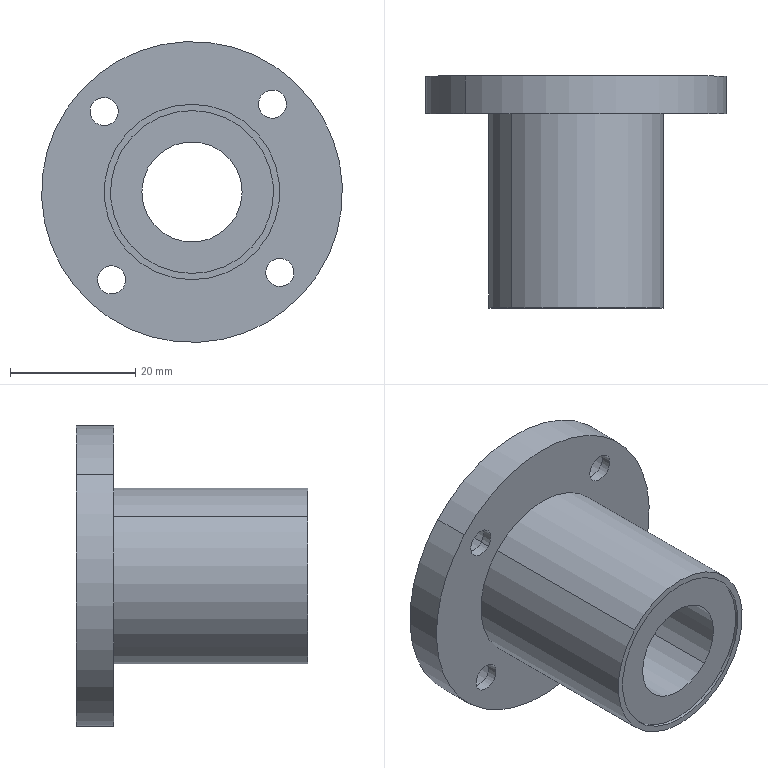Component | SolidWorks | LinearBearingSamickLMF16UU-5 | 1 solid | 38 faces | box 48 x 37 x 48 mm | volume 21132 mm3 | cylinder 28 | plane 10 | commonest cylinder face diameters 4.5 x8 8 x8 28 x4 26 x4 48 x2 16 x2
STEP:
#1=COLOUR_RGB('',0.7922,0.8196,0.9333);
#2=FILL_AREA_STYLE_COLOUR('',#1);
#3=FILL_AREA_STYLE('',(#2));
#4=SURFACE_STYLE_FILL_AREA(#3);
#5=SURFACE_SIDE_STYLE('',(#4));
#6=SURFACE_STYLE_USAGE(.BOTH.,#5);
#7=PRESENTATION_STYLE_ASSIGNMENT((#6));
#8=CARTESIAN_POINT('',(-6.706,-8.858,4.309));
#9=VERTEX_POINT('',#8);
#10=CARTESIAN_POINT('',(-5.893,-8.858,3.565));
#11=VERTEX_POINT('',#10);
#12=CARTESIAN_POINT('',(-6.299,-8.858,3.937));
#13=DIRECTION('',(0.,-1.,0.));
#14=DIRECTION('',(-0.7376,0.,0.6752));
#15=AXIS2_PLACEMENT_3D('',#12,#13,#14);
#16=CIRCLE('',#15,0.5512);
#17=EDGE_CURVE('',#9,#11,#16,.T.);
#18=ORIENTED_EDGE('',*,*,#17,.T.);
#19=CARTESIAN_POINT('',(-5.893,-10.079,3.565));
#20=VERTEX_POINT('',#19);
#21=CARTESIAN_POINT('',(-5.893,-8.622,3.565));
#22=DIRECTION('',(0.,-1.,0.));
#23=VECTOR('',#22,39.37);
#24=LINE('',#21,#23);
#25=EDGE_CURVE('',#11,#20,#24,.T.);
#26=ORIENTED_EDGE('',*,*,#25,.T.);
#27=CARTESIAN_POINT('',(-6.706,-10.079,4.309));
#28=VERTEX_POINT('',#27);
#29=CARTESIAN_POINT('',(-6.299,-10.079,3.937));
#30=DIRECTION('',(0.,1.,0.));
#31=DIRECTION('',(-0.7376,0.,0.6752));
#32=AXIS2_PLACEMENT_3D('',#29,#30,#31);
#33=CIRCLE('',#32,0.5512);
#34=EDGE_CURVE('',#20,#28,#33,.T.);
#35=ORIENTED_EDGE('',*,*,#34,.T.);
#36=CARTESIAN_POINT('',(-6.706,-8.622,4.309));
#37=DIRECTION('',(0.,-1.,0.));
#38=VECTOR('',#37,39.37);
#39=LINE('',#36,#38);
#40=EDGE_CURVE('',#9,#28,#39,.T.);
#41=ORIENTED_EDGE('',*,*,#40,.F.);
#42=EDGE_LOOP('',(#18,#26,#35,#41));
#43=FACE_OUTER_BOUND('',#42,.T.);
#44=CARTESIAN_POINT('',(-6.299,-8.622,3.937));
#45=DIRECTION('',(0.,-1.,0.));
#46=DIRECTION('',(-0.7376,0.,0.6752));
#47=AXIS2_PLACEMENT_3D('',#44,#45,#46);
#48=CYLINDRICAL_SURFACE('',#47,0.5512);
#49=ADVANCED_FACE('',(#43),#48,.T.);
#50=CARTESIAN_POINT('',(-5.922,-10.079,3.591));
#51=VERTEX_POINT('',#50);
#52=CARTESIAN_POINT('',(-6.677,-10.079,4.283));
#53=VERTEX_POINT('',#52);
#54=CARTESIAN_POINT('',(-6.299,-10.079,3.937));
#55=DIRECTION('',(0.,-1.,0.));
#56=DIRECTION('',(0.7376,0.,-0.6752));
#57=AXIS2_PLACEMENT_3D('',#54,#55,#56);
#58=CIRCLE('',#57,0.5118);
#59=EDGE_CURVE('',#51,#53,#58,.T.);
#60=ORIENTED_EDGE('',*,*,#59,.T.);
#61=CARTESIAN_POINT('',(-6.677,-10.059,4.283));
#62=VERTEX_POINT('',#61);
#63=CARTESIAN_POINT('',(-6.677,-10.079,4.283));
#64=DIRECTION('',(0.,1.,0.));
#65=VECTOR('',#64,39.37);
#66=LINE('',#63,#65);
#67=EDGE_CURVE('',#53,#62,#66,.T.);
#68=ORIENTED_EDGE('',*,*,#67,.T.);
#69=CARTESIAN_POINT('',(-5.922,-10.059,3.591));
#70=VERTEX_POINT('',#69);
#71=CARTESIAN_POINT('',(-6.299,-10.059,3.937));
#72=DIRECTION('',(0.,-1.,0.));
#73=DIRECTION('',(0.7376,0.,-0.6752));
#74=AXIS2_PLACEMENT_3D('',#71,#72,#73);
#75=CIRCLE('',#74,0.5118);
#76=EDGE_CURVE('',#70,#62,#75,.T.);
#77=ORIENTED_EDGE('',*,*,#76,.F.);
#78=CARTESIAN_POINT('',(-5.922,-10.079,3.591));
#79=DIRECTION('',(0.,1.,0.));
#80=VECTOR('',#79,39.37);
#81=LINE('',#78,#80);
#82=EDGE_CURVE('',#51,#70,#81,.T.);
#83=ORIENTED_EDGE('',*,*,#82,.F.);
#84=EDGE_LOOP('',(#60,#68,#77,#83));
#85=FACE_OUTER_BOUND('',#84,.T.);
#86=CARTESIAN_POINT('',(-6.299,-10.079,3.937));
#87=DIRECTION('',(0.,1.,0.));
#88=DIRECTION('',(0.7376,0.,-0.6752));
#89=AXIS2_PLACEMENT_3D('',#86,#87,#88);
#90=CYLINDRICAL_SURFACE('',#89,0.5118);
#91=ADVANCED_FACE('',(#85),#90,.F.);
#92=CARTESIAN_POINT('',(-6.864,-8.858,3.32));
#93=VERTEX_POINT('',#92);
#94=CARTESIAN_POINT('',(-6.744,-8.858,3.451));
#95=VERTEX_POINT('',#94);
#96=CARTESIAN_POINT('',(-6.804,-8.858,3.385));
#97=DIRECTION('',(0.,-1.,0.));
#98=DIRECTION('',(-0.6752,0.,-0.7376));
#99=AXIS2_PLACEMENT_3D('',#96,#97,#98);
#100=CIRCLE('',#99,0.08858);
#101=EDGE_CURVE('',#93,#95,#100,.T.);
#102=ORIENTED_EDGE('',*,*,#101,.T.);
#103=CARTESIAN_POINT('',(-6.744,-8.795,3.451));
#104=VERTEX_POINT('',#103);
#105=CARTESIAN_POINT('',(-6.744,-8.827,3.451));
#106=DIRECTION('',(-0.,1.,-0.));
#107=VECTOR('',#106,39.37);
#108=LINE('',#105,#107);
#109=EDGE_CURVE('',#95,#104,#108,.T.);
#110=ORIENTED_EDGE('',*,*,#109,.T.);
#111=CARTESIAN_POINT('',(-6.864,-8.795,3.32));
#112=VERTEX_POINT('',#111);
#113=CARTESIAN_POINT('',(-6.804,-8.795,3.385));
#114=DIRECTION('',(0.,-1.,0.));
#115=DIRECTION('',(-0.6752,0.,-0.7376));
#116=AXIS2_PLACEMENT_3D('',#113,#114,#115);
#117=CIRCLE('',#116,0.08858);
#118=EDGE_CURVE('',#112,#104,#117,.T.);
#119=ORIENTED_EDGE('',*,*,#118,.F.);
#120=CARTESIAN_POINT('',(-6.864,-8.827,3.32));
#121=DIRECTION('',(-0.,1.,-0.));
#122=VECTOR('',#121,39.37);
#123=LINE('',#120,#122);
#124=EDGE_CURVE('',#93,#112,#123,.T.);
#125=ORIENTED_EDGE('',*,*,#124,.F.);
#126=EDGE_LOOP('',(#102,#110,#119,#125));
#127=FACE_OUTER_BOUND('',#126,.T.);
#128=CARTESIAN_POINT('',(-6.804,-8.827,3.385));
#129=DIRECTION('',(-0.,1.,-0.));
#130=DIRECTION('',(-0.6752,0.,-0.7376));
#131=AXIS2_PLACEMENT_3D('',#128,#129,#130);
#132=CYLINDRICAL_SURFACE('',#131,0.08858);
#133=ADVANCED_FACE('',(#127),#132,.F.);
#134=CARTESIAN_POINT('',(-5.682,-8.858,3.372));
#135=VERTEX_POINT('',#134);
#136=CARTESIAN_POINT('',(-5.813,-8.858,3.492));
#137=VERTEX_POINT('',#136);
#138=CARTESIAN_POINT('',(-5.747,-8.858,3.432));
#139=DIRECTION('',(-0.,-1.,0.));
#140=DIRECTION('',(0.7376,0.,-0.6752));
#141=AXIS2_PLACEMENT_3D('',#138,#139,#140);
#142=CIRCLE('',#141,0.08858);
#143=EDGE_CURVE('',#135,#137,#142,.T.);
#144=ORIENTED_EDGE('',*,*,#143,.T.);
#145=CARTESIAN_POINT('',(-5.813,-8.795,3.492));
#146=VERTEX_POINT('',#145);
#147=CARTESIAN_POINT('',(-5.813,-8.827,3.492));
#148=DIRECTION('',(0.,1.,-0.));
#149=VECTOR('',#148,39.37);
#150=LINE('',#147,#149);
#151=EDGE_CURVE('',#137,#146,#150,.T.);
#152=ORIENTED_EDGE('',*,*,#151,.T.);
#153=CARTESIAN_POINT('',(-5.682,-8.795,3.372));
#154=VERTEX_POINT('',#153);
#155=CARTESIAN_POINT('',(-5.747,-8.795,3.432));
#156=DIRECTION('',(-0.,-1.,0.));
#157=DIRECTION('',(0.7376,0.,-0.6752));
#158=AXIS2_PLACEMENT_3D('',#155,#156,#157);
#159=CIRCLE('',#158,0.08858);
#160=EDGE_CURVE('',#154,#146,#159,.T.);
#161=ORIENTED_EDGE('',*,*,#160,.F.);
#162=CARTESIAN_POINT('',(-5.682,-8.827,3.372));
#163=DIRECTION('',(0.,1.,-0.));
#164=VECTOR('',#163,39.37);
#165=LINE('',#162,#164);
#166=EDGE_CURVE('',#135,#154,#165,.T.);
#167=ORIENTED_EDGE('',*,*,#166,.F.);
#168=EDGE_LOOP('',(#144,#152,#161,#167));
#169=FACE_OUTER_BOUND('',#168,.T.);
#170=CARTESIAN_POINT('',(-5.747,-8.827,3.432));
#171=DIRECTION('',(0.,1.,-0.));
#172=DIRECTION('',(0.7376,0.,-0.6752));
#173=AXIS2_PLACEMENT_3D('',#170,#171,#172);
#174=CYLINDRICAL_SURFACE('',#173,0.08858);
#175=ADVANCED_FACE('',(#169),#174,.F.);
#176=CARTESIAN_POINT('',(-5.854,-8.858,4.423));
#177=VERTEX_POINT('',#176);
#178=CARTESIAN_POINT('',(-5.734,-8.858,4.554));
#179=VERTEX_POINT('',#178);
#180=CARTESIAN_POINT('',(-5.794,-8.858,4.489));
#181=DIRECTION('',(-0.,-1.,-0.));
#182=DIRECTION('',(-0.6752,0.,-0.7376));
#183=AXIS2_PLACEMENT_3D('',#180,#181,#182);
#184=CIRCLE('',#183,0.08858);
#185=EDGE_CURVE('',#177,#179,#184,.T.);
#186=ORIENTED_EDGE('',*,*,#185,.T.);
#187=CARTESIAN_POINT('',(-5.734,-8.795,4.554));
#188=VERTEX_POINT('',#187);
#189=CARTESIAN_POINT('',(-5.734,-8.827,4.554));
#190=DIRECTION('',(0.,1.,0.));
#191=VECTOR('',#190,39.37);
#192=LINE('',#189,#191);
#193=EDGE_CURVE('',#179,#188,#192,.T.);
#194=ORIENTED_EDGE('',*,*,#193,.T.);
#195=CARTESIAN_POINT('',(-5.854,-8.795,4.423));
#196=VERTEX_POINT('',#195);
#197=CARTESIAN_POINT('',(-5.794,-8.795,4.489));
#198=DIRECTION('',(-0.,-1.,-0.));
#199=DIRECTION('',(-0.6752,0.,-0.7376));
#200=AXIS2_PLACEMENT_3D('',#197,#198,#199);
#201=CIRCLE('',#200,0.08858);
#202=EDGE_CURVE('',#196,#188,#201,.T.);
#203=ORIENTED_EDGE('',*,*,#202,.F.);
#204=CARTESIAN_POINT('',(-5.854,-8.827,4.423));
#205=DIRECTION('',(0.,1.,0.));
#206=VECTOR('',#205,39.37);
#207=LINE('',#204,#206);
#208=EDGE_CURVE('',#177,#196,#207,.T.);
#209=ORIENTED_EDGE('',*,*,#208,.F.);
#210=EDGE_LOOP('',(#186,#194,#203,#209));
#211=FACE_OUTER_BOUND('',#210,.T.);
#212=CARTESIAN_POINT('',(-5.794,-8.827,4.489));
#213=DIRECTION('',(0.,1.,0.));
#214=DIRECTION('',(-0.6752,0.,-0.7376));
#215=AXIS2_PLACEMENT_3D('',#212,#213,#214);
#216=CYLINDRICAL_SURFACE('',#215,0.08858);
#217=ADVANCED_FACE('',(#211),#216,.F.);
#218=CARTESIAN_POINT('',(-6.786,-8.858,4.382));
#219=VERTEX_POINT('',#218);
#220=CARTESIAN_POINT('',(-6.916,-8.858,4.502));
#221=VERTEX_POINT('',#220);
#222=CARTESIAN_POINT('',(-6.851,-8.858,4.442));
#223=DIRECTION('',(0.,-1.,-0.));
#224=DIRECTION('',(0.7376,0.,-0.6752));
#225=AXIS2_PLACEMENT_3D('',#222,#223,#224);
#226=CIRCLE('',#225,0.08858);
#227=EDGE_CURVE('',#219,#221,#226,.T.);
#228=ORIENTED_EDGE('',*,*,#227,.T.);
#229=CARTESIAN_POINT('',(-6.916,-8.795,4.502));
#230=VERTEX_POINT('',#229);
#231=CARTESIAN_POINT('',(-6.916,-8.827,4.502));
#232=DIRECTION('',(-0.,1.,0.));
#233=VECTOR('',#232,39.37);
#234=LINE('',#231,#233);
#235=EDGE_CURVE('',#221,#230,#234,.T.);
#236=ORIENTED_EDGE('',*,*,#235,.T.);
#237=CARTESIAN_POINT('',(-6.786,-8.795,4.382));
#238=VERTEX_POINT('',#237);
#239=CARTESIAN_POINT('',(-6.851,-8.795,4.442));
#240=DIRECTION('',(0.,-1.,-0.));
#241=DIRECTION('',(0.7376,0.,-0.6752));
#242=AXIS2_PLACEMENT_3D('',#239,#240,#241);
#243=CIRCLE('',#242,0.08858);
#244=EDGE_CURVE('',#238,#230,#243,.T.);
#245=ORIENTED_EDGE('',*,*,#244,.F.);
#246=CARTESIAN_POINT('',(-6.786,-8.827,4.382));
#247=DIRECTION('',(-0.,1.,0.));
#248=VECTOR('',#247,39.37);
#249=LINE('',#246,#248);
#250=EDGE_CURVE('',#219,#238,#249,.T.);
#251=ORIENTED_EDGE('',*,*,#250,.F.);
#252=EDGE_LOOP('',(#228,#236,#245,#251));
#253=FACE_OUTER_BOUND('',#252,.T.);
#254=CARTESIAN_POINT('',(-6.851,-8.827,4.442));
#255=DIRECTION('',(-0.,1.,0.));
#256=DIRECTION('',(0.7376,0.,-0.6752));
#257=AXIS2_PLACEMENT_3D('',#254,#255,#256);
#258=CYLINDRICAL_SURFACE('',#257,0.08858);
#259=ADVANCED_FACE('',(#253),#258,.F.);
#260=CARTESIAN_POINT('',(-6.996,-8.622,4.575));
#261=VERTEX_POINT('',#260);
#262=CARTESIAN_POINT('',(-5.602,-8.622,3.299));
#263=VERTEX_POINT('',#262);
#264=CARTESIAN_POINT('',(-6.299,-8.622,3.937));
#265=DIRECTION('',(0.,-1.,0.));
#266=DIRECTION('',(-0.7376,0.,0.6752));
#267=AXIS2_PLACEMENT_3D('',#264,#265,#266);
#268=CIRCLE('',#267,0.9449);
#269=EDGE_CURVE('',#261,#263,#268,.T.);
#270=ORIENTED_EDGE('',*,*,#269,.T.);
#271=CARTESIAN_POINT('',(-5.602,-8.858,3.299));
#272=VERTEX_POINT('',#271);
#273=CARTESIAN_POINT('',(-5.602,-8.622,3.299));
#274=DIRECTION('',(0.,-1.,0.));
#275=VECTOR('',#274,39.37);
#276=LINE('',#273,#275);
#277=EDGE_CURVE('',#263,#272,#276,.T.);
#278=ORIENTED_EDGE('',*,*,#277,.T.);
#279=CARTESIAN_POINT('',(-6.996,-8.858,4.575));
#280=VERTEX_POINT('',#279);
#281=CARTESIAN_POINT('',(-6.299,-8.858,3.937));
#282=DIRECTION('',(0.,1.,0.));
#283=DIRECTION('',(-0.7376,0.,0.6752));
#284=AXIS2_PLACEMENT_3D('',#281,#282,#283);
#285=CIRCLE('',#284,0.9449);
#286=EDGE_CURVE('',#272,#280,#285,.T.);
#287=ORIENTED_EDGE('',*,*,#286,.T.);
#288=CARTESIAN_POINT('',(-6.996,-8.622,4.575));
#289=DIRECTION('',(0.,-1.,0.));
#290=VECTOR('',#289,39.37);
#291=LINE('',#288,#290);
#292=EDGE_CURVE('',#261,#280,#291,.T.);
#293=ORIENTED_EDGE('',*,*,#292,.F.);
#294=EDGE_LOOP('',(#270,#278,#287,#293));
#295=FACE_OUTER_BOUND('',#294,.T.);
#296=CARTESIAN_POINT('',(-6.299,-8.622,3.937));
#297=DIRECTION('',(0.,-1.,0.));
#298=DIRECTION('',(-0.7376,0.,0.6752));
#299=AXIS2_PLACEMENT_3D('',#296,#297,#298);
#300=CYLINDRICAL_SURFACE('',#299,0.9449);
#301=ADVANCED_FACE('',(#295),#300,.T.);
#302=CARTESIAN_POINT('',(-6.067,-8.646,3.724));
#303=VERTEX_POINT('',#302);
#304=CARTESIAN_POINT('',(-6.532,-8.646,4.15));
#305=VERTEX_POINT('',#304);
#306=CARTESIAN_POINT('',(-6.299,-8.646,3.937));
#307=DIRECTION('',(0.,-1.,0.));
#308=DIRECTION('',(-0.7376,0.,0.6752));
#309=AXIS2_PLACEMENT_3D('',#306,#307,#308);
#310=CIRCLE('',#309,0.315);
#311=EDGE_CURVE('',#303,#305,#310,.T.);
#312=ORIENTED_EDGE('',*,*,#311,.F.);
#313=CARTESIAN_POINT('',(-6.067,-10.059,3.724));
#314=VERTEX_POINT('',#313);
#315=CARTESIAN_POINT('',(-6.067,-8.622,3.724));
#316=DIRECTION('',(0.,-1.,0.));
#317=VECTOR('',#316,39.37);
#318=LINE('',#315,#317);
#319=EDGE_CURVE('',#303,#314,#318,.T.);
#320=ORIENTED_EDGE('',*,*,#319,.T.);
#321=CARTESIAN_POINT('',(-6.532,-10.059,4.15));
#322=VERTEX_POINT('',#321);
#323=CARTESIAN_POINT('',(-6.299,-10.059,3.937));
#324=DIRECTION('',(0.,-1.,0.));
#325=DIRECTION('',(-0.7376,0.,0.6752));
#326=AXIS2_PLACEMENT_3D('',#323,#324,#325);
#327=CIRCLE('',#326,0.315);
#328=EDGE_CURVE('',#314,#322,#327,.T.);
#329=ORIENTED_EDGE('',*,*,#328,.T.);
#330=CARTESIAN_POINT('',(-6.532,-8.622,4.15));
#331=DIRECTION('',(0.,-1.,0.));
#332=VECTOR('',#331,39.37);
#333=LINE('',#330,#332);
#334=EDGE_CURVE('',#305,#322,#333,.T.);
#335=ORIENTED_EDGE('',*,*,#334,.F.);
#336=EDGE_LOOP('',(#312,#320,#329,#335));
#337=FACE_OUTER_BOUND('',#336,.T.);
#338=CARTESIAN_POINT('',(-6.299,-8.622,3.937));
#339=DIRECTION('',(0.,-1.,0.));
#340=DIRECTION('',(-0.7376,0.,0.6752));
#341=AXIS2_PLACEMENT_3D('',#338,#339,#340);
#342=CYLINDRICAL_SURFACE('',#341,0.315);
#343=ADVANCED_FACE('',(#337),#342,.F.);
#344=CARTESIAN_POINT('',(-6.911,-8.795,3.269));
#345=VERTEX_POINT('',#344);
#346=CARTESIAN_POINT('',(-6.698,-8.795,3.501));
#347=VERTEX_POINT('',#346);
#348=CARTESIAN_POINT('',(-6.804,-8.795,3.385));
#349=DIRECTION('',(0.,-1.,0.));
#350=DIRECTION('',(-0.6752,0.,-0.7376));
#351=AXIS2_PLACEMENT_3D('',#348,#349,#350);
#352=CIRCLE('',#351,0.1575);
#353=EDGE_CURVE('',#345,#347,#352,.T.);
#354=ORIENTED_EDGE('',*,*,#353,.T.);
#355=CARTESIAN_POINT('',(-6.698,-8.622,3.501));
#356=VERTEX_POINT('',#355);
#357=CARTESIAN_POINT('',(-6.698,-8.709,3.501));
#358=DIRECTION('',(-0.,1.,-0.));
#359=VECTOR('',#358,39.37);
#360=LINE('',#357,#359);
#361=EDGE_CURVE('',#347,#356,#360,.T.);
#362=ORIENTED_EDGE('',*,*,#361,.T.);
#363=CARTESIAN_POINT('',(-6.911,-8.622,3.269));
#364=VERTEX_POINT('',#363);
#365=CARTESIAN_POINT('',(-6.804,-8.622,3.385));
#366=DIRECTION('',(0.,-1.,0.));
#367=DIRECTION('',(-0.6752,0.,-0.7376));
#368=AXIS2_PLACEMENT_3D('',#365,#366,#367);
#369=CIRCLE('',#368,0.1575);
#370=EDGE_CURVE('',#364,#356,#369,.T.);
#371=ORIENTED_EDGE('',*,*,#370,.F.);
#372=CARTESIAN_POINT('',(-6.911,-8.709,3.269));
#373=DIRECTION('',(-0.,1.,-0.));
#374=VECTOR('',#373,39.37);
#375=LINE('',#372,#374);
#376=EDGE_CURVE('',#345,#364,#375,.T.);
#377=ORIENTED_EDGE('',*,*,#376,.F.);
#378=EDGE_LOOP('',(#354,#362,#371,#377));
#379=FACE_OUTER_BOUND('',#378,.T.);
#380=CARTESIAN_POINT('',(-6.804,-8.709,3.385));
#381=DIRECTION('',(-0.,1.,-0.));
#382=DIRECTION('',(-0.6752,0.,-0.7376));
#383=AXIS2_PLACEMENT_3D('',#380,#381,#382);
#384=CYLINDRICAL_SURFACE('',#383,0.1575);
#385=ADVANCED_FACE('',(#379),#384,.F.);
#386=CARTESIAN_POINT('',(-5.631,-8.795,3.326));
#387=VERTEX_POINT('',#386);
#388=CARTESIAN_POINT('',(-5.864,-8.795,3.538));
#389=VERTEX_POINT('',#388);
#390=CARTESIAN_POINT('',(-5.747,-8.795,3.432));
#391=DIRECTION('',(-0.,-1.,0.));
#392=DIRECTION('',(0.7376,0.,-0.6752));
#393=AXIS2_PLACEMENT_3D('',#390,#391,#392);
#394=CIRCLE('',#393,0.1575);
#395=EDGE_CURVE('',#387,#389,#394,.T.);
#396=ORIENTED_EDGE('',*,*,#395,.T.);
#397=CARTESIAN_POINT('',(-5.864,-8.622,3.538));
#398=VERTEX_POINT('',#397);
#399=CARTESIAN_POINT('',(-5.864,-8.709,3.538));
#400=DIRECTION('',(0.,1.,-0.));
#401=VECTOR('',#400,39.37);
#402=LINE('',#399,#401);
#403=EDGE_CURVE('',#389,#398,#402,.T.);
#404=ORIENTED_EDGE('',*,*,#403,.T.);
#405=CARTESIAN_POINT('',(-5.631,-8.622,3.326));
#406=VERTEX_POINT('',#405);
#407=CARTESIAN_POINT('',(-5.747,-8.622,3.432));
#408=DIRECTION('',(-0.,-1.,0.));
#409=DIRECTION('',(0.7376,0.,-0.6752));
#410=AXIS2_PLACEMENT_3D('',#407,#408,#409);
#411=CIRCLE('',#410,0.1575);
#412=EDGE_CURVE('',#406,#398,#411,.T.);
#413=ORIENTED_EDGE('',*,*,#412,.F.);
#414=CARTESIAN_POINT('',(-5.631,-8.709,3.326));
#415=DIRECTION('',(0.,1.,-0.));
#416=VECTOR('',#415,39.37);
#417=LINE('',#414,#416);
#418=EDGE_CURVE('',#387,#406,#417,.T.);
#419=ORIENTED_EDGE('',*,*,#418,.F.);
#420=EDGE_LOOP('',(#396,#404,#413,#419));
#421=FACE_OUTER_BOUND('',#420,.T.);
#422=CARTESIAN_POINT('',(-5.747,-8.709,3.432));
#423=DIRECTION('',(0.,1.,-0.));
#424=DIRECTION('',(0.7376,0.,-0.6752));
#425=AXIS2_PLACEMENT_3D('',#422,#423,#424);
#426=CYLINDRICAL_SURFACE('',#425,0.1575);
#427=ADVANCED_FACE('',(#421),#426,.F.);
#428=CARTESIAN_POINT('',(-5.9,-8.795,4.373));
#429=VERTEX_POINT('',#428);
#430=CARTESIAN_POINT('',(-5.688,-8.795,4.605));
#431=VERTEX_POINT('',#430);
#432=CARTESIAN_POINT('',(-5.794,-8.795,4.489));
#433=DIRECTION('',(-0.,-1.,-0.));
#434=DIRECTION('',(-0.6752,0.,-0.7376));
#435=AXIS2_PLACEMENT_3D('',#432,#433,#434);
#436=CIRCLE('',#435,0.1575);
#437=EDGE_CURVE('',#429,#431,#436,.T.);
#438=ORIENTED_EDGE('',*,*,#437,.T.);
#439=CARTESIAN_POINT('',(-5.688,-8.622,4.605));
#440=VERTEX_POINT('',#439);
#441=CARTESIAN_POINT('',(-5.688,-8.709,4.605));
#442=DIRECTION('',(0.,1.,0.));
#443=VECTOR('',#442,39.37);
#444=LINE('',#441,#443);
#445=EDGE_CURVE('',#431,#440,#444,.T.);
#446=ORIENTED_EDGE('',*,*,#445,.T.);
#447=CARTESIAN_POINT('',(-5.9,-8.622,4.373));
#448=VERTEX_POINT('',#447);
#449=CARTESIAN_POINT('',(-5.794,-8.622,4.489));
#450=DIRECTION('',(-0.,-1.,-0.));
#451=DIRECTION('',(-0.6752,0.,-0.7376));
#452=AXIS2_PLACEMENT_3D('',#449,#450,#451);
#453=CIRCLE('',#452,0.1575);
#454=EDGE_CURVE('',#448,#440,#453,.T.);
#455=ORIENTED_EDGE('',*,*,#454,.F.);
#456=CARTESIAN_POINT('',(-5.9,-8.709,4.373));
#457=DIRECTION('',(0.,1.,0.));
#458=VECTOR('',#457,39.37);
#459=LINE('',#456,#458);
#460=EDGE_CURVE('',#429,#448,#459,.T.);
#461=ORIENTED_EDGE('',*,*,#460,.F.);
#462=EDGE_LOOP('',(#438,#446,#455,#461));
#463=FACE_OUTER_BOUND('',#462,.T.);
#464=CARTESIAN_POINT('',(-5.794,-8.709,4.489));
#465=DIRECTION('',(0.,1.,0.));
#466=DIRECTION('',(-0.6752,0.,-0.7376));
#467=AXIS2_PLACEMENT_3D('',#464,#465,#466);
#468=CYLINDRICAL_SURFACE('',#467,0.1575);
#469=ADVANCED_FACE('',(#463),#468,.F.);
#470=CARTESIAN_POINT('',(-6.735,-8.795,4.336));
#471=VERTEX_POINT('',#470);
#472=CARTESIAN_POINT('',(-6.967,-8.795,4.548));
#473=VERTEX_POINT('',#472);
#474=CARTESIAN_POINT('',(-6.851,-8.795,4.442));
#475=DIRECTION('',(0.,-1.,-0.));
#476=DIRECTION('',(0.7376,0.,-0.6752));
#477=AXIS2_PLACEMENT_3D('',#474,#475,#476);
#478=CIRCLE('',#477,0.1575);
#479=EDGE_CURVE('',#471,#473,#478,.T.);
#480=ORIENTED_EDGE('',*,*,#479,.T.);
#481=CARTESIAN_POINT('',(-6.967,-8.622,4.548));
#482=VERTEX_POINT('',#481);
#483=CARTESIAN_POINT('',(-6.967,-8.709,4.548));
#484=DIRECTION('',(-0.,1.,0.));
#485=VECTOR('',#484,39.37);
#486=LINE('',#483,#485);
#487=EDGE_CURVE('',#473,#482,#486,.T.);
#488=ORIENTED_EDGE('',*,*,#487,.T.);
#489=CARTESIAN_POINT('',(-6.735,-8.622,4.336));
#490=VERTEX_POINT('',#489);
#491=CARTESIAN_POINT('',(-6.851,-8.622,4.442));
#492=DIRECTION('',(0.,-1.,-0.));
#493=DIRECTION('',(0.7376,0.,-0.6752));
#494=AXIS2_PLACEMENT_3D('',#491,#492,#493);
#495=CIRCLE('',#494,0.1575);
#496=EDGE_CURVE('',#490,#482,#495,.T.);
#497=ORIENTED_EDGE('',*,*,#496,.F.);
#498=CARTESIAN_POINT('',(-6.735,-8.709,4.336));
#499=DIRECTION('',(-0.,1.,0.));
#500=VECTOR('',#499,39.37);
#501=LINE('',#498,#500);
#502=EDGE_CURVE('',#471,#490,#501,.T.);
#503=ORIENTED_EDGE('',*,*,#502,.F.);
#504=EDGE_LOOP('',(#480,#488,#497,#503));
#505=FACE_OUTER_BOUND('',#504,.T.);
#506=CARTESIAN_POINT('',(-6.851,-8.709,4.442));
#507=DIRECTION('',(-0.,1.,0.));
#508=DIRECTION('',(0.7376,0.,-0.6752));
#509=AXIS2_PLACEMENT_3D('',#506,#507,#508);
#510=CYLINDRICAL_SURFACE('',#509,0.1575);
#511=ADVANCED_FACE('',(#505),#510,.F.);
#512=CARTESIAN_POINT('',(-5.893,-8.622,3.565));
#513=VERTEX_POINT('',#512);
#514=CARTESIAN_POINT('',(-6.706,-8.622,4.309));
#515=VERTEX_POINT('',#514);
#516=CARTESIAN_POINT('',(-6.299,-8.622,3.937));
#517=DIRECTION('',(0.,-1.,0.));
#518=DIRECTION('',(-0.7376,0.,0.6752));
#519=AXIS2_PLACEMENT_3D('',#516,#517,#518);
#520=CIRCLE('',#519,0.5512);
#521=EDGE_CURVE('',#513,#515,#520,.T.);
#522=ORIENTED_EDGE('',*,*,#521,.F.);
#523=CARTESIAN_POINT('',(-5.893,-8.634,3.565));
#524=VERTEX_POINT('',#523);
#525=CARTESIAN_POINT('',(-5.893,-8.622,3.565));
#526=DIRECTION('',(0.,-1.,0.));
#527=VECTOR('',#526,39.37);
#528=LINE('',#525,#527);
#529=EDGE_CURVE('',#513,#524,#528,.T.);
#530=ORIENTED_EDGE('',*,*,#529,.T.);
#531=CARTESIAN_POINT('',(-6.706,-8.634,4.309));
#532=VERTEX_POINT('',#531);
#533=CARTESIAN_POINT('',(-6.299,-8.634,3.937));
#534=DIRECTION('',(0.,1.,0.));
#535=DIRECTION('',(-0.7376,0.,0.6752));
#536=AXIS2_PLACEMENT_3D('',#533,#534,#535);
#537=CIRCLE('',#536,0.5512);
#538=EDGE_CURVE('',#532,#524,#537,.T.);
#539=ORIENTED_EDGE('',*,*,#538,.F.);
#540=CARTESIAN_POINT('',(-6.706,-8.622,4.309));
#541=DIRECTION('',(0.,-1.,0.));
#542=VECTOR('',#541,39.37);
#543=LINE('',#540,#542);
#544=EDGE_CURVE('',#515,#532,#543,.T.);
#545=ORIENTED_EDGE('',*,*,#544,.F.);
#546=EDGE_LOOP('',(#522,#530,#539,#545));
#547=FACE_OUTER_BOUND('',#546,.T.);
#548=CARTESIAN_POINT('',(-6.299,-8.622,3.937));
#549=DIRECTION('',(0.,-1.,0.));
#550=DIRECTION('',(-0.7376,0.,0.6752));
#551=AXIS2_PLACEMENT_3D('',#548,#549,#550);
#552=CYLINDRICAL_SURFACE('',#551,0.5512);
#553=ADVANCED_FACE('',(#547),#552,.F.);
#554=CARTESIAN_POINT('',(-5.922,-8.634,3.591));
#555=VERTEX_POINT('',#554);
#556=CARTESIAN_POINT('',(-6.677,-8.634,4.283));
#557=VERTEX_POINT('',#556);
#558=CARTESIAN_POINT('',(-6.299,-8.634,3.937));
#559=DIRECTION('',(0.,-1.,0.));
#560=DIRECTION('',(-0.7376,0.,0.6752));
#561=AXIS2_PLACEMENT_3D('',#558,#559,#560);
#562=CIRCLE('',#561,0.5118);
#563=EDGE_CURVE('',#555,#557,#562,.T.);
#564=ORIENTED_EDGE('',*,*,#563,.F.);
#565=CARTESIAN_POINT('',(-5.922,-8.646,3.591));
#566=VERTEX_POINT('',#565);
#567=CARTESIAN_POINT('',(-5.922,-8.622,3.591));
#568=DIRECTION('',(0.,-1.,0.));
#569=VECTOR('',#568,39.37);
#570=LINE('',#567,#569);
#571=EDGE_CURVE('',#555,#566,#570,.T.);
#572=ORIENTED_EDGE('',*,*,#571,.T.);
#573=CARTESIAN_POINT('',(-6.677,-8.646,4.283));
#574=VERTEX_POINT('',#573);
#575=CARTESIAN_POINT('',(-6.299,-8.646,3.937));
#576=DIRECTION('',(0.,1.,0.));
#577=DIRECTION('',(-0.7376,0.,0.6752));
#578=AXIS2_PLACEMENT_3D('',#575,#576,#577);
#579=CIRCLE('',#578,0.5118);
#580=EDGE_CURVE('',#574,#566,#579,.T.);
#581=ORIENTED_EDGE('',*,*,#580,.F.);
#582=CARTESIAN_POINT('',(-6.677,-8.622,4.283));
#583=DIRECTION('',(0.,-1.,0.));
#584=VECTOR('',#583,39.37);
#585=LINE('',#582,#584);
#586=EDGE_CURVE('',#557,#574,#585,.T.);
#587=ORIENTED_EDGE('',*,*,#586,.F.);
#588=EDGE_LOOP('',(#564,#572,#581,#587));
#589=FACE_OUTER_BOUND('',#588,.T.);
#590=CARTESIAN_POINT('',(-6.299,-8.622,3.937));
#591=DIRECTION('',(0.,-1.,0.));
#592=DIRECTION('',(-0.7376,0.,0.6752));
#593=AXIS2_PLACEMENT_3D('',#590,#591,#592);
#594=CYLINDRICAL_SURFACE('',#593,0.5118);
#595=ADVANCED_FACE('',(#589),#594,.F.);
#596=ORIENTED_EDGE('',*,*,#25,.F.);
#597=CARTESIAN_POINT('',(-6.299,-8.858,3.937));
#598=DIRECTION('',(0.,-1.,0.));
#599=DIRECTION('',(-0.7376,0.,0.6752));
#600=AXIS2_PLACEMENT_3D('',#597,#598,#599);
#601=CIRCLE('',#600,0.5512);
#602=EDGE_CURVE('',#11,#9,#601,.T.);
#603=ORIENTED_EDGE('',*,*,#602,.T.);
#604=ORIENTED_EDGE('',*,*,#40,.T.);
#605=CARTESIAN_POINT('',(-6.299,-10.079,3.937));
#606=DIRECTION('',(0.,1.,0.));
#607=DIRECTION('',(-0.7376,0.,0.6752));
#608=AXIS2_PLACEMENT_3D('',#605,#606,#607);
#609=CIRCLE('',#608,0.5512);
#610=EDGE_CURVE('',#28,#20,#609,.T.);
#611=ORIENTED_EDGE('',*,*,#610,.T.);
#612=EDGE_LOOP('',(#596,#603,#604,#611));
#613=FACE_OUTER_BOUND('',#612,.T.);
#614=CARTESIAN_POINT('',(-6.299,-8.622,3.937));
#615=DIRECTION('',(0.,-1.,0.));
#616=DIRECTION('',(-0.7376,0.,0.6752));
#617=AXIS2_PLACEMENT_3D('',#614,#615,#616);
#618=CYLINDRICAL_SURFACE('',#617,0.5512);
#619=ADVANCED_FACE('',(#613),#618,.T.);
#620=ORIENTED_EDGE('',*,*,#59,.F.);
#621=CARTESIAN_POINT('',(-6.299,-10.079,3.937));
#622=DIRECTION('',(0.,-1.,0.));
#623=DIRECTION('',(0.7376,0.,-0.6752));
#624=AXIS2_PLACEMENT_3D('',#621,#622,#623);
#625=CIRCLE('',#624,0.5118);
#626=EDGE_CURVE('',#53,#51,#625,.T.);
#627=ORIENTED_EDGE('',*,*,#626,.F.);
#628=EDGE_LOOP('',(#620,#627));
#629=FACE_BOUND('',#628,.T.);
#630=ORIENTED_EDGE('',*,*,#610,.F.);
#631=ORIENTED_EDGE('',*,*,#34,.F.);
#632=EDGE_LOOP('',(#630,#631));
#633=FACE_OUTER_BOUND('',#632,.T.);
#634=CARTESIAN_POINT('',(-6.299,-10.079,3.937));
#635=DIRECTION('',(0.,1.,0.));
#636=DIRECTION('',(0.7376,0.,-0.6752));
#637=AXIS2_PLACEMENT_3D('',#634,#635,#636);
#638=PLANE('',#637);
#639=ADVANCED_FACE('',(#629,#633),#638,.F.);
#640=ORIENTED_EDGE('',*,*,#17,.F.);
#641=ORIENTED_EDGE('',*,*,#602,.F.);
#642=EDGE_LOOP('',(#640,#641));
#643=FACE_BOUND('',#642,.T.);
#644=ORIENTED_EDGE('',*,*,#101,.F.);
#645=CARTESIAN_POINT('',(-6.804,-8.858,3.385));
#646=DIRECTION('',(0.,-1.,0.));
#647=DIRECTION('',(-0.6752,0.,-0.7376));
#648=AXIS2_PLACEMENT_3D('',#645,#646,#647);
#649=CIRCLE('',#648,0.08858);
#650=EDGE_CURVE('',#95,#93,#649,.T.);
#651=ORIENTED_EDGE('',*,*,#650,.F.);
#652=EDGE_LOOP('',(#644,#651));
#653=FACE_BOUND('',#652,.T.);
#654=ORIENTED_EDGE('',*,*,#143,.F.);
#655=CARTESIAN_POINT('',(-5.747,-8.858,3.432));
#656=DIRECTION('',(-0.,-1.,0.));
#657=DIRECTION('',(0.7376,0.,-0.6752));
#658=AXIS2_PLACEMENT_3D('',#655,#656,#657);
#659=CIRCLE('',#658,0.08858);
#660=EDGE_CURVE('',#137,#135,#659,.T.);
#661=ORIENTED_EDGE('',*,*,#660,.F.);
#662=EDGE_LOOP('',(#654,#661));
#663=FACE_BOUND('',#662,.T.);
#664=ORIENTED_EDGE('',*,*,#185,.F.);
#665=CARTESIAN_POINT('',(-5.794,-8.858,4.489));
#666=DIRECTION('',(-0.,-1.,-0.));
#667=DIRECTION('',(-0.6752,0.,-0.7376));
#668=AXIS2_PLACEMENT_3D('',#665,#666,#667);
#669=CIRCLE('',#668,0.08858);
#670=EDGE_CURVE('',#179,#177,#669,.T.);
#671=ORIENTED_EDGE('',*,*,#670,.F.);
#672=EDGE_LOOP('',(#664,#671));
#673=FACE_BOUND('',#672,.T.);
#674=ORIENTED_EDGE('',*,*,#227,.F.);
#675=CARTESIAN_POINT('',(-6.851,-8.858,4.442));
#676=DIRECTION('',(0.,-1.,-0.));
#677=DIRECTION('',(0.7376,0.,-0.6752));
#678=AXIS2_PLACEMENT_3D('',#675,#676,#677);
#679=CIRCLE('',#678,0.08858);
#680=EDGE_CURVE('',#221,#219,#679,.T.);
#681=ORIENTED_EDGE('',*,*,#680,.F.);
#682=EDGE_LOOP('',(#674,#681));
#683=FACE_BOUND('',#682,.T.);
#684=CARTESIAN_POINT('',(-6.299,-8.858,3.937));
#685=DIRECTION('',(0.,1.,0.));
#686=DIRECTION('',(-0.7376,0.,0.6752));
#687=AXIS2_PLACEMENT_3D('',#684,#685,#686);
#688=CIRCLE('',#687,0.9449);
#689=EDGE_CURVE('',#280,#272,#688,.T.);
#690=ORIENTED_EDGE('',*,*,#689,.F.);
#691=ORIENTED_EDGE('',*,*,#286,.F.);
#692=EDGE_LOOP('',(#690,#691));
#693=FACE_OUTER_BOUND('',#692,.T.);
#694=CARTESIAN_POINT('',(-6.299,-8.858,3.937));
#695=DIRECTION('',(0.,1.,0.));
#696=DIRECTION('',(0.7376,0.,-0.6752));
#697=AXIS2_PLACEMENT_3D('',#694,#695,#696);
#698=PLANE('',#697);
#699=ADVANCED_FACE('',(#643,#653,#663,#673,#683,#693),#698,.F.);
#700=ORIENTED_EDGE('',*,*,#67,.F.);
#701=ORIENTED_EDGE('',*,*,#626,.T.);
#702=ORIENTED_EDGE('',*,*,#82,.T.);
#703=CARTESIAN_POINT('',(-6.299,-10.059,3.937));
#704=DIRECTION('',(0.,-1.,0.));
#705=DIRECTION('',(0.7376,0.,-0.6752));
#706=AXIS2_PLACEMENT_3D('',#703,#704,#705);
#707=CIRCLE('',#706,0.5118);
#708=EDGE_CURVE('',#62,#70,#707,.T.);
#709=ORIENTED_EDGE('',*,*,#708,.F.);
#710=EDGE_LOOP('',(#700,#701,#702,#709));
#711=FACE_OUTER_BOUND('',#710,.T.);
#712=CARTESIAN_POINT('',(-6.299,-10.079,3.937));
#713=DIRECTION('',(0.,1.,0.));
#714=DIRECTION('',(0.7376,0.,-0.6752));
#715=AXIS2_PLACEMENT_3D('',#712,#713,#714);
#716=CYLINDRICAL_SURFACE('',#715,0.5118);
#717=ADVANCED_FACE('',(#711),#716,.F.);
#718=ORIENTED_EDGE('',*,*,#109,.F.);
#719=ORIENTED_EDGE('',*,*,#650,.T.);
#720=ORIENTED_EDGE('',*,*,#124,.T.);
#721=CARTESIAN_POINT('',(-6.804,-8.795,3.385));
#722=DIRECTION('',(0.,-1.,0.));
#723=DIRECTION('',(-0.6752,0.,-0.7376));
#724=AXIS2_PLACEMENT_3D('',#721,#722,#723);
#725=CIRCLE('',#724,0.08858);
#726=EDGE_CURVE('',#104,#112,#725,.T.);
#727=ORIENTED_EDGE('',*,*,#726,.F.);
#728=EDGE_LOOP('',(#718,#719,#720,#727));
#729=FACE_OUTER_BOUND('',#728,.T.);
#730=CARTESIAN_POINT('',(-6.804,-8.827,3.385));
#731=DIRECTION('',(-0.,1.,-0.));
#732=DIRECTION('',(-0.6752,0.,-0.7376));
#733=AXIS2_PLACEMENT_3D('',#730,#731,#732);
#734=CYLINDRICAL_SURFACE('',#733,0.08858);
#735=ADVANCED_FACE('',(#729),#734,.F.);
#736=ORIENTED_EDGE('',*,*,#151,.F.);
#737=ORIENTED_EDGE('',*,*,#660,.T.);
#738=ORIENTED_EDGE('',*,*,#166,.T.);
#739=CARTESIAN_POINT('',(-5.747,-8.795,3.432));
#740=DIRECTION('',(-0.,-1.,0.));
#741=DIRECTION('',(0.7376,0.,-0.6752));
#742=AXIS2_PLACEMENT_3D('',#739,#740,#741);
#743=CIRCLE('',#742,0.08858);
#744=EDGE_CURVE('',#146,#154,#743,.T.);
#745=ORIENTED_EDGE('',*,*,#744,.F.);
#746=EDGE_LOOP('',(#736,#737,#738,#745));
#747=FACE_OUTER_BOUND('',#746,.T.);
#748=CARTESIAN_POINT('',(-5.747,-8.827,3.432));
#749=DIRECTION('',(0.,1.,-0.));
#750=DIRECTION('',(0.7376,0.,-0.6752));
#751=AXIS2_PLACEMENT_3D('',#748,#749,#750);
#752=CYLINDRICAL_SURFACE('',#751,0.08858);
#753=ADVANCED_FACE('',(#747),#752,.F.);
#754=ORIENTED_EDGE('',*,*,#193,.F.);
#755=ORIENTED_EDGE('',*,*,#670,.T.);
#756=ORIENTED_EDGE('',*,*,#208,.T.);
#757=CARTESIAN_POINT('',(-5.794,-8.795,4.489));
#758=DIRECTION('',(-0.,-1.,-0.));
#759=DIRECTION('',(-0.6752,0.,-0.7376));
#760=AXIS2_PLACEMENT_3D('',#757,#758,#759);
#761=CIRCLE('',#760,0.08858);
#762=EDGE_CURVE('',#188,#196,#761,.T.);
#763=ORIENTED_EDGE('',*,*,#762,.F.);
#764=EDGE_LOOP('',(#754,#755,#756,#763));
#765=FACE_OUTER_BOUND('',#764,.T.);
#766=CARTESIAN_POINT('',(-5.794,-8.827,4.489));
#767=DIRECTION('',(0.,1.,0.));
#768=DIRECTION('',(-0.6752,0.,-0.7376));
#769=AXIS2_PLACEMENT_3D('',#766,#767,#768);
#770=CYLINDRICAL_SURFACE('',#769,0.08858);
#771=ADVANCED_FACE('',(#765),#770,.F.);
#772=ORIENTED_EDGE('',*,*,#235,.F.);
#773=ORIENTED_EDGE('',*,*,#680,.T.);
#774=ORIENTED_EDGE('',*,*,#250,.T.);
#775=CARTESIAN_POINT('',(-6.851,-8.795,4.442));
#776=DIRECTION('',(0.,-1.,-0.));
#777=DIRECTION('',(0.7376,0.,-0.6752));
#778=AXIS2_PLACEMENT_3D('',#775,#776,#777);
#779=CIRCLE('',#778,0.08858);
#780=EDGE_CURVE('',#230,#238,#779,.T.);
#781=ORIENTED_EDGE('',*,*,#780,.F.);
#782=EDGE_LOOP('',(#772,#773,#774,#781));
#783=FACE_OUTER_BOUND('',#782,.T.);
#784=CARTESIAN_POINT('',(-6.851,-8.827,4.442));
#785=DIRECTION('',(-0.,1.,0.));
#786=DIRECTION('',(0.7376,0.,-0.6752));
#787=AXIS2_PLACEMENT_3D('',#784,#785,#786);
#788=CYLINDRICAL_SURFACE('',#787,0.08858);
#789=ADVANCED_FACE('',(#783),#788,.F.);
#790=ORIENTED_EDGE('',*,*,#277,.F.);
#791=CARTESIAN_POINT('',(-6.299,-8.622,3.937));
#792=DIRECTION('',(0.,-1.,0.));
#793=DIRECTION('',(-0.7376,0.,0.6752));
#794=AXIS2_PLACEMENT_3D('',#791,#792,#793);
#795=CIRCLE('',#794,0.9449);
#796=EDGE_CURVE('',#263,#261,#795,.T.);
#797=ORIENTED_EDGE('',*,*,#796,.T.);
#798=ORIENTED_EDGE('',*,*,#292,.T.);
#799=ORIENTED_EDGE('',*,*,#689,.T.);
#800=EDGE_LOOP('',(#790,#797,#798,#799));
#801=FACE_OUTER_BOUND('',#800,.T.);
#802=CARTESIAN_POINT('',(-6.299,-8.622,3.937));
#803=DIRECTION('',(0.,-1.,0.));
#804=DIRECTION('',(-0.7376,0.,0.6752));
#805=AXIS2_PLACEMENT_3D('',#802,#803,#804);
#806=CYLINDRICAL_SURFACE('',#805,0.9449);
#807=ADVANCED_FACE('',(#801),#806,.T.);
#808=CARTESIAN_POINT('',(-6.299,-10.059,3.937));
#809=DIRECTION('',(0.,-1.,0.));
#810=DIRECTION('',(-0.7376,0.,0.6752));
#811=AXIS2_PLACEMENT_3D('',#808,#809,#810);
#812=CIRCLE('',#811,0.315);
#813=EDGE_CURVE('',#322,#314,#812,.T.);
#814=ORIENTED_EDGE('',*,*,#813,.F.);
#815=ORIENTED_EDGE('',*,*,#328,.F.);
#816=EDGE_LOOP('',(#814,#815));
#817=FACE_BOUND('',#816,.T.);
#818=ORIENTED_EDGE('',*,*,#76,.T.);
#819=ORIENTED_EDGE('',*,*,#708,.T.);
#820=EDGE_LOOP('',(#818,#819));
#821=FACE_OUTER_BOUND('',#820,.T.);
#822=CARTESIAN_POINT('',(-6.299,-10.059,3.937));
#823=DIRECTION('',(0.,1.,0.));
#824=DIRECTION('',(0.7376,0.,-0.6752));
#825=AXIS2_PLACEMENT_3D('',#822,#823,#824);
#826=PLANE('',#825);
#827=ADVANCED_FACE('',(#817,#821),#826,.F.);
#828=ORIENTED_EDGE('',*,*,#118,.T.);
#829=ORIENTED_EDGE('',*,*,#726,.T.);
#830=EDGE_LOOP('',(#828,#829));
#831=FACE_BOUND('',#830,.T.);
#832=ORIENTED_EDGE('',*,*,#353,.F.);
#833=CARTESIAN_POINT('',(-6.804,-8.795,3.385));
#834=DIRECTION('',(0.,-1.,0.));
#835=DIRECTION('',(-0.6752,0.,-0.7376));
#836=AXIS2_PLACEMENT_3D('',#833,#834,#835);
#837=CIRCLE('',#836,0.1575);
#838=EDGE_CURVE('',#347,#345,#837,.T.);
#839=ORIENTED_EDGE('',*,*,#838,.F.);
#840=EDGE_LOOP('',(#832,#839));
#841=FACE_OUTER_BOUND('',#840,.T.);
#842=CARTESIAN_POINT('',(-6.721,-8.795,3.476));
#843=DIRECTION('',(0.,-1.,0.));
#844=DIRECTION('',(-0.7376,0.,0.6752));
#845=AXIS2_PLACEMENT_3D('',#842,#843,#844);
#846=PLANE('',#845);
#847=ADVANCED_FACE('',(#831,#841),#846,.F.);
#848=ORIENTED_EDGE('',*,*,#160,.T.);
#849=ORIENTED_EDGE('',*,*,#744,.T.);
#850=EDGE_LOOP('',(#848,#849));
#851=FACE_BOUND('',#850,.T.);
#852=ORIENTED_EDGE('',*,*,#395,.F.);
#853=CARTESIAN_POINT('',(-5.747,-8.795,3.432));
#854=DIRECTION('',(-0.,-1.,0.));
#855=DIRECTION('',(0.7376,0.,-0.6752));
#856=AXIS2_PLACEMENT_3D('',#853,#854,#855);
#857=CIRCLE('',#856,0.1575);
#858=EDGE_CURVE('',#389,#387,#857,.T.);
#859=ORIENTED_EDGE('',*,*,#858,.F.);
#860=EDGE_LOOP('',(#852,#859));
#861=FACE_OUTER_BOUND('',#860,.T.);
#862=CARTESIAN_POINT('',(-5.838,-8.795,3.515));
#863=DIRECTION('',(0.,-1.,0.));
#864=DIRECTION('',(-0.7376,0.,0.6752));
#865=AXIS2_PLACEMENT_3D('',#862,#863,#864);
#866=PLANE('',#865);
#867=ADVANCED_FACE('',(#851,#861),#866,.F.);
#868=ORIENTED_EDGE('',*,*,#202,.T.);
#869=ORIENTED_EDGE('',*,*,#762,.T.);
#870=EDGE_LOOP('',(#868,#869));
#871=FACE_BOUND('',#870,.T.);
#872=ORIENTED_EDGE('',*,*,#437,.F.);
#873=CARTESIAN_POINT('',(-5.794,-8.795,4.489));
#874=DIRECTION('',(-0.,-1.,-0.));
#875=DIRECTION('',(-0.6752,0.,-0.7376));
#876=AXIS2_PLACEMENT_3D('',#873,#874,#875);
#877=CIRCLE('',#876,0.1575);
#878=EDGE_CURVE('',#431,#429,#877,.T.);
#879=ORIENTED_EDGE('',*,*,#878,.F.);
#880=EDGE_LOOP('',(#872,#879));
#881=FACE_OUTER_BOUND('',#880,.T.);
#882=CARTESIAN_POINT('',(-5.877,-8.795,4.398));
#883=DIRECTION('',(0.,-1.,0.));
#884=DIRECTION('',(-0.7376,0.,0.6752));
#885=AXIS2_PLACEMENT_3D('',#882,#883,#884);
#886=PLANE('',#885);
#887=ADVANCED_FACE('',(#871,#881),#886,.F.);
#888=ORIENTED_EDGE('',*,*,#244,.T.);
#889=ORIENTED_EDGE('',*,*,#780,.T.);
#890=EDGE_LOOP('',(#888,#889));
#891=FACE_BOUND('',#890,.T.);
#892=ORIENTED_EDGE('',*,*,#479,.F.);
#893=CARTESIAN_POINT('',(-6.851,-8.795,4.442));
#894=DIRECTION('',(0.,-1.,-0.));
#895=DIRECTION('',(0.7376,0.,-0.6752));
#896=AXIS2_PLACEMENT_3D('',#893,#894,#895);
#897=CIRCLE('',#896,0.1575);
#898=EDGE_CURVE('',#473,#471,#897,.T.);
#899=ORIENTED_EDGE('',*,*,#898,.F.);
#900=EDGE_LOOP('',(#892,#899));
#901=FACE_OUTER_BOUND('',#900,.T.);
#902=CARTESIAN_POINT('',(-6.76,-8.795,4.359));
#903=DIRECTION('',(0.,-1.,0.));
#904=DIRECTION('',(-0.7376,0.,0.6752));
#905=AXIS2_PLACEMENT_3D('',#902,#903,#904);
#906=PLANE('',#905);
#907=ADVANCED_FACE('',(#891,#901),#906,.F.);
#908=CARTESIAN_POINT('',(-6.299,-8.622,3.937));
#909=DIRECTION('',(0.,-1.,0.));
#910=DIRECTION('',(-0.7376,0.,0.6752));
#911=AXIS2_PLACEMENT_3D('',#908,#909,#910);
#912=CIRCLE('',#911,0.5512);
#913=EDGE_CURVE('',#515,#513,#912,.T.);
#914=ORIENTED_EDGE('',*,*,#913,.T.);
#915=ORIENTED_EDGE('',*,*,#521,.T.);
#916=EDGE_LOOP('',(#914,#915));
#917=FACE_BOUND('',#916,.T.);
#918=ORIENTED_EDGE('',*,*,#370,.T.);
#919=CARTESIAN_POINT('',(-6.804,-8.622,3.385));
#920=DIRECTION('',(0.,-1.,0.));
#921=DIRECTION('',(-0.6752,0.,-0.7376));
#922=AXIS2_PLACEMENT_3D('',#919,#920,#921);
#923=CIRCLE('',#922,0.1575);
#924=EDGE_CURVE('',#356,#364,#923,.T.);
#925=ORIENTED_EDGE('',*,*,#924,.T.);
#926=EDGE_LOOP('',(#918,#925));
#927=FACE_BOUND('',#926,.T.);
#928=ORIENTED_EDGE('',*,*,#412,.T.);
#929=CARTESIAN_POINT('',(-5.747,-8.622,3.432));
#930=DIRECTION('',(-0.,-1.,0.));
#931=DIRECTION('',(0.7376,0.,-0.6752));
#932=AXIS2_PLACEMENT_3D('',#929,#930,#931);
#933=CIRCLE('',#932,0.1575);
#934=EDGE_CURVE('',#398,#406,#933,.T.);
#935=ORIENTED_EDGE('',*,*,#934,.T.);
#936=EDGE_LOOP('',(#928,#935));
#937=FACE_BOUND('',#936,.T.);
#938=ORIENTED_EDGE('',*,*,#454,.T.);
#939=CARTESIAN_POINT('',(-5.794,-8.622,4.489));
#940=DIRECTION('',(-0.,-1.,-0.));
#941=DIRECTION('',(-0.6752,0.,-0.7376));
#942=AXIS2_PLACEMENT_3D('',#939,#940,#941);
#943=CIRCLE('',#942,0.1575);
#944=EDGE_CURVE('',#440,#448,#943,.T.);
#945=ORIENTED_EDGE('',*,*,#944,.T.);
#946=EDGE_LOOP('',(#938,#945));
#947=FACE_BOUND('',#946,.T.);
#948=ORIENTED_EDGE('',*,*,#496,.T.);
#949=CARTESIAN_POINT('',(-6.851,-8.622,4.442));
#950=DIRECTION('',(0.,-1.,-0.));
#951=DIRECTION('',(0.7376,0.,-0.6752));
#952=AXIS2_PLACEMENT_3D('',#949,#950,#951);
#953=CIRCLE('',#952,0.1575);
#954=EDGE_CURVE('',#482,#490,#953,.T.);
#955=ORIENTED_EDGE('',*,*,#954,.T.);
#956=EDGE_LOOP('',(#948,#955));
#957=FACE_BOUND('',#956,.T.);
#958=ORIENTED_EDGE('',*,*,#269,.F.);
#959=ORIENTED_EDGE('',*,*,#796,.F.);
#960=EDGE_LOOP('',(#958,#959));
#961=FACE_OUTER_BOUND('',#960,.T.);
#962=CARTESIAN_POINT('',(-6.299,-8.622,3.937));
#963=DIRECTION('',(0.,1.,0.));
#964=DIRECTION('',(0.7376,0.,-0.6752));
#965=AXIS2_PLACEMENT_3D('',#962,#963,#964);
#966=PLANE('',#965);
#967=ADVANCED_FACE('',(#917,#927,#937,#947,#957,#961),#966,.T.);
#968=ORIENTED_EDGE('',*,*,#319,.F.);
#969=CARTESIAN_POINT('',(-6.299,-8.646,3.937));
#970=DIRECTION('',(0.,-1.,0.));
#971=DIRECTION('',(-0.7376,0.,0.6752));
#972=AXIS2_PLACEMENT_3D('',#969,#970,#971);
#973=CIRCLE('',#972,0.315);
#974=EDGE_CURVE('',#305,#303,#973,.T.);
#975=ORIENTED_EDGE('',*,*,#974,.F.);
#976=ORIENTED_EDGE('',*,*,#334,.T.);
#977=ORIENTED_EDGE('',*,*,#813,.T.);
#978=EDGE_LOOP('',(#968,#975,#976,#977));
#979=FACE_OUTER_BOUND('',#978,.T.);
#980=CARTESIAN_POINT('',(-6.299,-8.622,3.937));
#981=DIRECTION('',(0.,-1.,0.));
#982=DIRECTION('',(-0.7376,0.,0.6752));
#983=AXIS2_PLACEMENT_3D('',#980,#981,#982);
#984=CYLINDRICAL_SURFACE('',#983,0.315);
#985=ADVANCED_FACE('',(#979),#984,.F.);
#986=ORIENTED_EDGE('',*,*,#361,.F.);
#987=ORIENTED_EDGE('',*,*,#838,.T.);
#988=ORIENTED_EDGE('',*,*,#376,.T.);
#989=ORIENTED_EDGE('',*,*,#924,.F.);
#990=EDGE_LOOP('',(#986,#987,#988,#989));
#991=FACE_OUTER_BOUND('',#990,.T.);
#992=CARTESIAN_POINT('',(-6.804,-8.709,3.385));
#993=DIRECTION('',(-0.,1.,-0.));
#994=DIRECTION('',(-0.6752,0.,-0.7376));
#995=AXIS2_PLACEMENT_3D('',#992,#993,#994);
#996=CYLINDRICAL_SURFACE('',#995,0.1575);
#997=ADVANCED_FACE('',(#991),#996,.F.);
#998=ORIENTED_EDGE('',*,*,#403,.F.);
#999=ORIENTED_EDGE('',*,*,#858,.T.);
#1000=ORIENTED_EDGE('',*,*,#418,.T.);
#1001=ORIENTED_EDGE('',*,*,#934,.F.);
#1002=EDGE_LOOP('',(#998,#999,#1000,#1001));
#1003=FACE_OUTER_BOUND('',#1002,.T.);
#1004=CARTESIAN_POINT('',(-5.747,-8.709,3.432));
#1005=DIRECTION('',(0.,1.,-0.));
#1006=DIRECTION('',(0.7376,0.,-0.6752));
#1007=AXIS2_PLACEMENT_3D('',#1004,#1005,#1006);
#1008=CYLINDRICAL_SURFACE('',#1007,0.1575);
#1009=ADVANCED_FACE('',(#1003),#1008,.F.);
#1010=ORIENTED_EDGE('',*,*,#445,.F.);
#1011=ORIENTED_EDGE('',*,*,#878,.T.);
#1012=ORIENTED_EDGE('',*,*,#460,.T.);
#1013=ORIENTED_EDGE('',*,*,#944,.F.);
#1014=EDGE_LOOP('',(#1010,#1011,#1012,#1013));
#1015=FACE_OUTER_BOUND('',#1014,.T.);
#1016=CARTESIAN_POINT('',(-5.794,-8.709,4.489));
#1017=DIRECTION('',(0.,1.,0.));
#1018=DIRECTION('',(-0.6752,0.,-0.7376));
#1019=AXIS2_PLACEMENT_3D('',#1016,#1017,#1018);
#1020=CYLINDRICAL_SURFACE('',#1019,0.1575);
#1021=ADVANCED_FACE('',(#1015),#1020,.F.);
#1022=ORIENTED_EDGE('',*,*,#487,.F.);
#1023=ORIENTED_EDGE('',*,*,#898,.T.);
#1024=ORIENTED_EDGE('',*,*,#502,.T.);
#1025=ORIENTED_EDGE('',*,*,#954,.F.);
#1026=EDGE_LOOP('',(#1022,#1023,#1024,#1025));
#1027=FACE_OUTER_BOUND('',#1026,.T.);
#1028=CARTESIAN_POINT('',(-6.851,-8.709,4.442));
#1029=DIRECTION('',(-0.,1.,0.));
#1030=DIRECTION('',(0.7376,0.,-0.6752));
#1031=AXIS2_PLACEMENT_3D('',#1028,#1029,#1030);
#1032=CYLINDRICAL_SURFACE('',#1031,0.1575);
#1033=ADVANCED_FACE('',(#1027),#1032,.F.);
#1034=ORIENTED_EDGE('',*,*,#529,.F.);
#1035=ORIENTED_EDGE('',*,*,#913,.F.);
#1036=ORIENTED_EDGE('',*,*,#544,.T.);
#1037=CARTESIAN_POINT('',(-6.299,-8.634,3.937));
#1038=DIRECTION('',(0.,1.,0.));
#1039=DIRECTION('',(-0.7376,0.,0.6752));
#1040=AXIS2_PLACEMENT_3D('',#1037,#1038,#1039);
#1041=CIRCLE('',#1040,0.5512);
#1042=EDGE_CURVE('',#524,#532,#1041,.T.);
#1043=ORIENTED_EDGE('',*,*,#1042,.F.);
#1044=EDGE_LOOP('',(#1034,#1035,#1036,#1043));
#1045=FACE_OUTER_BOUND('',#1044,.T.);
#1046=CARTESIAN_POINT('',(-6.299,-8.622,3.937));
#1047=DIRECTION('',(0.,-1.,0.));
#1048=DIRECTION('',(-0.7376,0.,0.6752));
#1049=AXIS2_PLACEMENT_3D('',#1046,#1047,#1048);
#1050=CYLINDRICAL_SURFACE('',#1049,0.5512);
#1051=ADVANCED_FACE('',(#1045),#1050,.F.);
#1052=ORIENTED_EDGE('',*,*,#974,.T.);
#1053=ORIENTED_EDGE('',*,*,#311,.T.);
#1054=EDGE_LOOP('',(#1052,#1053));
#1055=FACE_BOUND('',#1054,.T.);
#1056=ORIENTED_EDGE('',*,*,#580,.T.);
#1057=CARTESIAN_POINT('',(-6.299,-8.646,3.937));
#1058=DIRECTION('',(0.,1.,0.));
#1059=DIRECTION('',(-0.7376,0.,0.6752));
#1060=AXIS2_PLACEMENT_3D('',#1057,#1058,#1059);
#1061=CIRCLE('',#1060,0.5118);
#1062=EDGE_CURVE('',#566,#574,#1061,.T.);
#1063=ORIENTED_EDGE('',*,*,#1062,.T.);
#1064=EDGE_LOOP('',(#1056,#1063));
#1065=FACE_OUTER_BOUND('',#1064,.T.);
#1066=CARTESIAN_POINT('',(-6.299,-8.646,3.937));
#1067=DIRECTION('',(0.,1.,0.));
#1068=DIRECTION('',(0.7376,0.,-0.6752));
#1069=AXIS2_PLACEMENT_3D('',#1066,#1067,#1068);
#1070=PLANE('',#1069);
#1071=ADVANCED_FACE('',(#1055,#1065),#1070,.T.);
#1072=CARTESIAN_POINT('',(-6.299,-8.634,3.937));
#1073=DIRECTION('',(0.,-1.,0.));
#1074=DIRECTION('',(-0.7376,0.,0.6752));
#1075=AXIS2_PLACEMENT_3D('',#1072,#1073,#1074);
#1076=CIRCLE('',#1075,0.5118);
#1077=EDGE_CURVE('',#557,#555,#1076,.T.);
#1078=ORIENTED_EDGE('',*,*,#1077,.T.);
#1079=ORIENTED_EDGE('',*,*,#563,.T.);
#1080=EDGE_LOOP('',(#1078,#1079));
#1081=FACE_BOUND('',#1080,.T.);
#1082=ORIENTED_EDGE('',*,*,#538,.T.);
#1083=ORIENTED_EDGE('',*,*,#1042,.T.);
#1084=EDGE_LOOP('',(#1082,#1083));
#1085=FACE_OUTER_BOUND('',#1084,.T.);
#1086=CARTESIAN_POINT('',(-6.299,-8.634,3.937));
#1087=DIRECTION('',(0.,1.,0.));
#1088=DIRECTION('',(0.7376,0.,-0.6752));
#1089=AXIS2_PLACEMENT_3D('',#1086,#1087,#1088);
#1090=PLANE('',#1089);
#1091=ADVANCED_FACE('',(#1081,#1085),#1090,.T.);
#1092=ORIENTED_EDGE('',*,*,#571,.F.);
#1093=ORIENTED_EDGE('',*,*,#1077,.F.);
#1094=ORIENTED_EDGE('',*,*,#586,.T.);
#1095=ORIENTED_EDGE('',*,*,#1062,.F.);
#1096=EDGE_LOOP('',(#1092,#1093,#1094,#1095));
#1097=FACE_OUTER_BOUND('',#1096,.T.);
#1098=CARTESIAN_POINT('',(-6.299,-8.622,3.937));
#1099=DIRECTION('',(0.,-1.,0.));
#1100=DIRECTION('',(-0.7376,0.,0.6752));
#1101=AXIS2_PLACEMENT_3D('',#1098,#1099,#1100);
#1102=CYLINDRICAL_SURFACE('',#1101,0.5118);
#1103=ADVANCED_FACE('',(#1097),#1102,.F.);
#1104=CLOSED_SHELL('',(#49,#91,#133,#175,#217,#259,#301,#343,#385,#427,#469,#511,#553,#595,#619,#639,#699,#717,#735,#753,#771,#789,#807,#827,#847,#867,#887,#907,#967,#985,#997,#1009,#1021,#1033,#1051,#1071,#1091,#1103));
#1105=MANIFOLD_SOLID_BREP('',#1104);
#1106=STYLED_ITEM('',(#7),#1105);
#1107=(LENGTH_UNIT()NAMED_UNIT(*)SI_UNIT($,.METRE.));
#1108=LENGTH_MEASURE_WITH_UNIT(LENGTH_MEASURE(0.0254),#1107);
#1109=DIMENSIONAL_EXPONENTS(1.,0.,0.,0.,0.,0.,0.);
#1110=(CONVERSION_BASED_UNIT('',#1108)LENGTH_UNIT()NAMED_UNIT(#1109));
#1111=UNCERTAINTY_MEASURE_WITH_UNIT(LENGTH_MEASURE(0.00001),#1110,'','');
#1112=(NAMED_UNIT(*)PLANE_ANGLE_UNIT()SI_UNIT($,.RADIAN.));
#1113=(NAMED_UNIT(*)SI_UNIT($,.STERADIAN.)SOLID_ANGLE_UNIT());
#1114=(GEOMETRIC_REPRESENTATION_CONTEXT(3)GLOBAL_UNCERTAINTY_ASSIGNED_CONTEXT((#1111))GLOBAL_UNIT_ASSIGNED_CONTEXT((#1110,#1112,#1113))REPRESENTATION_CONTEXT('',''));
#1115=MECHANICAL_DESIGN_GEOMETRIC_PRESENTATION_REPRESENTATION('',(#1106),#1114);
#1116=PRESENTATION_LAYER_ASSIGNMENT('','',(#1106));
#1117=CARTESIAN_POINT('',(0.,0.,0.));
#1118=DIRECTION('',(0.,0.,1.));
#1119=DIRECTION('',(1.,0.,0.));
#1120=AXIS2_PLACEMENT_3D('',#1117,#1118,#1119);
#1121=(LENGTH_UNIT()NAMED_UNIT(*)SI_UNIT($,.METRE.));
#1122=LENGTH_MEASURE_WITH_UNIT(LENGTH_MEASURE(0.0254),#1121);
#1123=DIMENSIONAL_EXPONENTS(1.,0.,0.,0.,0.,0.,0.);
#1124=(CONVERSION_BASED_UNIT('',#1122)LENGTH_UNIT()NAMED_UNIT(#1123));
#1125=UNCERTAINTY_MEASURE_WITH_UNIT(LENGTH_MEASURE(0.00001),#1124,'','');
#1126=(NAMED_UNIT(*)PLANE_ANGLE_UNIT()SI_UNIT($,.RADIAN.));
#1127=(NAMED_UNIT(*)SI_UNIT($,.STERADIAN.)SOLID_ANGLE_UNIT());
#1128=(GEOMETRIC_REPRESENTATION_CONTEXT(3)GLOBAL_UNCERTAINTY_ASSIGNED_CONTEXT((#1125))GLOBAL_UNIT_ASSIGNED_CONTEXT((#1124,#1126,#1127))REPRESENTATION_CONTEXT('',''));
#1129=ADVANCED_BREP_SHAPE_REPRESENTATION('',(#1105,#1120),#1128);